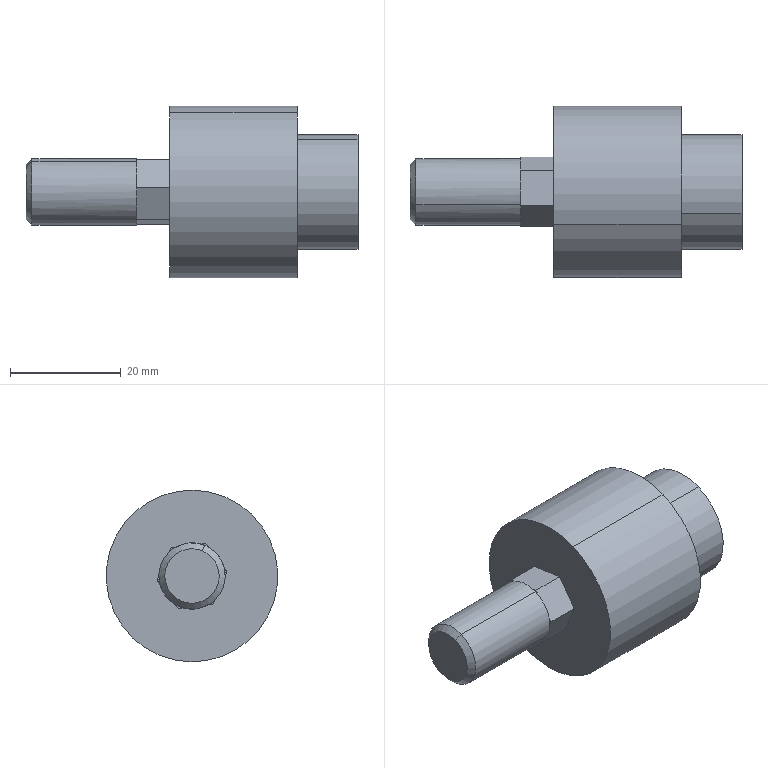Component | SolidWorks | FloatingJointSMCJA40-12-175-1 | 1 solid | 33 faces | box 60 x 31 x 31 mm | volume 22336 mm3 | plane 23 | cylinder 8 | cone 2 | commonest cylinder face diameters 12 x4 31 x2 20.667 x2
STEP:
#1=COLOUR_RGB('',0.7922,0.8196,0.9333);
#2=FILL_AREA_STYLE_COLOUR('',#1);
#3=FILL_AREA_STYLE('',(#2));
#4=SURFACE_STYLE_FILL_AREA(#3);
#5=SURFACE_SIDE_STYLE('',(#4));
#6=SURFACE_STYLE_USAGE(.BOTH.,#5);
#7=PRESENTATION_STYLE_ASSIGNMENT((#6));
#8=CARTESIAN_POINT('',(-1.88,0.09048,-0.2182));
#9=VERTEX_POINT('',#8);
#10=CARTESIAN_POINT('',(-1.88,-0.09048,0.2182));
#11=VERTEX_POINT('',#10);
#12=CARTESIAN_POINT('',(-1.88,-0.,0.));
#13=DIRECTION('',(1.,0.,-0.));
#14=DIRECTION('',(0.,-0.383,0.9237));
#15=AXIS2_PLACEMENT_3D('',#12,#13,#14);
#16=CIRCLE('',#15,0.2362);
#17=EDGE_CURVE('',#9,#11,#16,.T.);
#18=ORIENTED_EDGE('',*,*,#17,.T.);
#19=CARTESIAN_POINT('',(-2.431,-0.09048,0.2182));
#20=VERTEX_POINT('',#19);
#21=CARTESIAN_POINT('',(-1.329,-0.09048,0.2182));
#22=DIRECTION('',(-1.,-0.,0.));
#23=VECTOR('',#22,39.37);
#24=LINE('',#21,#23);
#25=EDGE_CURVE('',#11,#20,#24,.T.);
#26=ORIENTED_EDGE('',*,*,#25,.T.);
#27=CARTESIAN_POINT('',(-2.431,0.09048,-0.2182));
#28=VERTEX_POINT('',#27);
#29=CARTESIAN_POINT('',(-2.431,-0.,0.));
#30=DIRECTION('',(-1.,-0.,0.));
#31=DIRECTION('',(0.,0.383,-0.9237));
#32=AXIS2_PLACEMENT_3D('',#29,#30,#31);
#33=CIRCLE('',#32,0.2362);
#34=EDGE_CURVE('',#20,#28,#33,.T.);
#35=ORIENTED_EDGE('',*,*,#34,.T.);
#36=CARTESIAN_POINT('',(-1.329,0.09048,-0.2182));
#37=DIRECTION('',(-1.,-0.,0.));
#38=VECTOR('',#37,39.37);
#39=LINE('',#36,#38);
#40=EDGE_CURVE('',#9,#28,#39,.T.);
#41=ORIENTED_EDGE('',*,*,#40,.F.);
#42=EDGE_LOOP('',(#18,#26,#35,#41));
#43=FACE_OUTER_BOUND('',#42,.T.);
#44=CARTESIAN_POINT('',(-1.329,0.,-0.));
#45=DIRECTION('',(-1.,-0.,0.));
#46=DIRECTION('',(0.,0.383,-0.9237));
#47=AXIS2_PLACEMENT_3D('',#44,#45,#46);
#48=CYLINDRICAL_SURFACE('',#47,0.2362);
#49=ADVANCED_FACE('',(#43),#48,.F.);
#50=CARTESIAN_POINT('',(-3.219,-0.2338,0.5637));
#51=VERTEX_POINT('',#50);
#52=CARTESIAN_POINT('',(-3.219,0.2338,-0.5637));
#53=VERTEX_POINT('',#52);
#54=CARTESIAN_POINT('',(-3.219,-0.,0.));
#55=DIRECTION('',(1.,0.,-0.));
#56=DIRECTION('',(0.,-0.383,0.9237));
#57=AXIS2_PLACEMENT_3D('',#54,#55,#56);
#58=CIRCLE('',#57,0.6102);
#59=EDGE_CURVE('',#51,#53,#58,.T.);
#60=ORIENTED_EDGE('',*,*,#59,.T.);
#61=CARTESIAN_POINT('',(-2.313,0.2338,-0.5637));
#62=VERTEX_POINT('',#61);
#63=CARTESIAN_POINT('',(-2.766,0.2338,-0.5637));
#64=DIRECTION('',(1.,0.,-0.));
#65=VECTOR('',#64,39.37);
#66=LINE('',#63,#65);
#67=EDGE_CURVE('',#53,#62,#66,.T.);
#68=ORIENTED_EDGE('',*,*,#67,.T.);
#69=CARTESIAN_POINT('',(-2.313,-0.2338,0.5637));
#70=VERTEX_POINT('',#69);
#71=CARTESIAN_POINT('',(-2.313,-0.,0.));
#72=DIRECTION('',(-1.,-0.,0.));
#73=DIRECTION('',(0.,-0.383,0.9237));
#74=AXIS2_PLACEMENT_3D('',#71,#72,#73);
#75=CIRCLE('',#74,0.6102);
#76=EDGE_CURVE('',#62,#70,#75,.T.);
#77=ORIENTED_EDGE('',*,*,#76,.T.);
#78=CARTESIAN_POINT('',(-2.766,-0.2338,0.5637));
#79=DIRECTION('',(1.,0.,-0.));
#80=VECTOR('',#79,39.37);
#81=LINE('',#78,#80);
#82=EDGE_CURVE('',#51,#70,#81,.T.);
#83=ORIENTED_EDGE('',*,*,#82,.F.);
#84=EDGE_LOOP('',(#60,#68,#77,#83));
#85=FACE_OUTER_BOUND('',#84,.T.);
#86=CARTESIAN_POINT('',(-2.766,-0.,0.));
#87=DIRECTION('',(1.,0.,-0.));
#88=DIRECTION('',(0.,-0.383,0.9237));
#89=AXIS2_PLACEMENT_3D('',#86,#87,#88);
#90=CYLINDRICAL_SURFACE('',#89,0.6102);
#91=ADVANCED_FACE('',(#85),#90,.T.);
#92=CARTESIAN_POINT('',(-2.313,0.1558,-0.3758));
#93=VERTEX_POINT('',#92);
#94=CARTESIAN_POINT('',(-2.313,-0.1558,0.3758));
#95=VERTEX_POINT('',#94);
#96=CARTESIAN_POINT('',(-2.313,-0.,0.));
#97=DIRECTION('',(-1.,-0.,0.));
#98=DIRECTION('',(0.,-0.383,0.9237));
#99=AXIS2_PLACEMENT_3D('',#96,#97,#98);
#100=CIRCLE('',#99,0.4068);
#101=EDGE_CURVE('',#93,#95,#100,.T.);
#102=ORIENTED_EDGE('',*,*,#101,.F.);
#103=CARTESIAN_POINT('',(-1.88,0.1558,-0.3758));
#104=VERTEX_POINT('',#103);
#105=CARTESIAN_POINT('',(-2.096,0.1558,-0.3758));
#106=DIRECTION('',(1.,0.,-0.));
#107=VECTOR('',#106,39.37);
#108=LINE('',#105,#107);
#109=EDGE_CURVE('',#93,#104,#108,.T.);
#110=ORIENTED_EDGE('',*,*,#109,.T.);
#111=CARTESIAN_POINT('',(-1.88,-0.1558,0.3758));
#112=VERTEX_POINT('',#111);
#113=CARTESIAN_POINT('',(-1.88,-0.,0.));
#114=DIRECTION('',(-1.,-0.,0.));
#115=DIRECTION('',(0.,-0.383,0.9237));
#116=AXIS2_PLACEMENT_3D('',#113,#114,#115);
#117=CIRCLE('',#116,0.4068);
#118=EDGE_CURVE('',#104,#112,#117,.T.);
#119=ORIENTED_EDGE('',*,*,#118,.T.);
#120=CARTESIAN_POINT('',(-2.096,-0.1558,0.3758));
#121=DIRECTION('',(1.,0.,-0.));
#122=VECTOR('',#121,39.37);
#123=LINE('',#120,#122);
#124=EDGE_CURVE('',#95,#112,#123,.T.);
#125=ORIENTED_EDGE('',*,*,#124,.F.);
#126=EDGE_LOOP('',(#102,#110,#119,#125));
#127=FACE_OUTER_BOUND('',#126,.T.);
#128=CARTESIAN_POINT('',(-2.096,-0.,0.));
#129=DIRECTION('',(1.,0.,-0.));
#130=DIRECTION('',(0.,-0.383,0.9237));
#131=AXIS2_PLACEMENT_3D('',#128,#129,#130);
#132=CYLINDRICAL_SURFACE('',#131,0.4068);
#133=ADVANCED_FACE('',(#127),#132,.T.);
#134=CARTESIAN_POINT('',(-4.2,-0.09048,0.2182));
#135=VERTEX_POINT('',#134);
#136=CARTESIAN_POINT('',(-4.2,0.09048,-0.2182));
#137=VERTEX_POINT('',#136);
#138=CARTESIAN_POINT('',(-4.2,-0.,0.));
#139=DIRECTION('',(1.,0.,-0.));
#140=DIRECTION('',(0.,-0.383,0.9237));
#141=AXIS2_PLACEMENT_3D('',#138,#139,#140);
#142=CIRCLE('',#141,0.2362);
#143=EDGE_CURVE('',#135,#137,#142,.T.);
#144=ORIENTED_EDGE('',*,*,#143,.T.);
#145=CARTESIAN_POINT('',(-3.455,0.09048,-0.2182));
#146=VERTEX_POINT('',#145);
#147=CARTESIAN_POINT('',(-3.827,0.09048,-0.2182));
#148=DIRECTION('',(1.,0.,-0.));
#149=VECTOR('',#148,39.37);
#150=LINE('',#147,#149);
#151=EDGE_CURVE('',#137,#146,#150,.T.);
#152=ORIENTED_EDGE('',*,*,#151,.T.);
#153=CARTESIAN_POINT('',(-3.455,0.06542,-0.227));
#154=VERTEX_POINT('',#153);
#155=CARTESIAN_POINT('',(-3.455,-0.,0.));
#156=DIRECTION('',(1.,0.,-0.));
#157=DIRECTION('',(0.,-0.383,0.9237));
#158=AXIS2_PLACEMENT_3D('',#155,#156,#157);
#159=CIRCLE('',#158,0.2362);
#160=EDGE_CURVE('',#154,#146,#159,.T.);
#161=ORIENTED_EDGE('',*,*,#160,.F.);
#162=CARTESIAN_POINT('',(-3.455,-0.1218,-0.2024));
#163=VERTEX_POINT('',#162);
#164=CARTESIAN_POINT('',(-3.455,-0.,0.));
#165=DIRECTION('',(1.,0.,-0.));
#166=DIRECTION('',(0.,-0.383,0.9237));
#167=AXIS2_PLACEMENT_3D('',#164,#165,#166);
#168=CIRCLE('',#167,0.2362);
#169=EDGE_CURVE('',#163,#154,#168,.T.);
#170=ORIENTED_EDGE('',*,*,#169,.F.);
#171=CARTESIAN_POINT('',(-3.455,-0.1639,-0.1701));
#172=VERTEX_POINT('',#171);
#173=CARTESIAN_POINT('',(-3.455,-0.,0.));
#174=DIRECTION('',(1.,0.,-0.));
#175=DIRECTION('',(0.,-0.383,0.9237));
#176=AXIS2_PLACEMENT_3D('',#173,#174,#175);
#177=CIRCLE('',#176,0.2362);
#178=EDGE_CURVE('',#172,#163,#177,.T.);
#179=ORIENTED_EDGE('',*,*,#178,.F.);
#180=CARTESIAN_POINT('',(-3.455,-0.2362,0.004262));
#181=VERTEX_POINT('',#180);
#182=CARTESIAN_POINT('',(-3.455,-0.,0.));
#183=DIRECTION('',(1.,0.,-0.));
#184=DIRECTION('',(0.,-0.383,0.9237));
#185=AXIS2_PLACEMENT_3D('',#182,#183,#184);
#186=CIRCLE('',#185,0.2362);
#187=EDGE_CURVE('',#181,#172,#186,.T.);
#188=ORIENTED_EDGE('',*,*,#187,.F.);
#189=CARTESIAN_POINT('',(-3.455,-0.2293,0.05683));
#190=VERTEX_POINT('',#189);
#191=CARTESIAN_POINT('',(-3.455,-0.,0.));
#192=DIRECTION('',(1.,0.,-0.));
#193=DIRECTION('',(0.,-0.383,0.9237));
#194=AXIS2_PLACEMENT_3D('',#191,#192,#193);
#195=CIRCLE('',#194,0.2362);
#196=EDGE_CURVE('',#190,#181,#195,.T.);
#197=ORIENTED_EDGE('',*,*,#196,.F.);
#198=CARTESIAN_POINT('',(-3.455,-0.1144,0.2067));
#199=VERTEX_POINT('',#198);
#200=CARTESIAN_POINT('',(-3.455,-0.,0.));
#201=DIRECTION('',(1.,0.,-0.));
#202=DIRECTION('',(0.,-0.383,0.9237));
#203=AXIS2_PLACEMENT_3D('',#200,#201,#202);
#204=CIRCLE('',#203,0.2362);
#205=EDGE_CURVE('',#199,#190,#204,.T.);
#206=ORIENTED_EDGE('',*,*,#205,.F.);
#207=CARTESIAN_POINT('',(-3.455,-0.09048,0.2182));
#208=VERTEX_POINT('',#207);
#209=CARTESIAN_POINT('',(-3.455,-0.,0.));
#210=DIRECTION('',(1.,0.,-0.));
#211=DIRECTION('',(0.,-0.383,0.9237));
#212=AXIS2_PLACEMENT_3D('',#209,#210,#211);
#213=CIRCLE('',#212,0.2362);
#214=EDGE_CURVE('',#208,#199,#213,.T.);
#215=ORIENTED_EDGE('',*,*,#214,.F.);
#216=CARTESIAN_POINT('',(-3.827,-0.09048,0.2182));
#217=DIRECTION('',(1.,0.,-0.));
#218=VECTOR('',#217,39.37);
#219=LINE('',#216,#218);
#220=EDGE_CURVE('',#135,#208,#219,.T.);
#221=ORIENTED_EDGE('',*,*,#220,.F.);
#222=EDGE_LOOP('',(#144,#152,#161,#170,#179,#188,#197,#206,#215,#221));
#223=FACE_OUTER_BOUND('',#222,.T.);
#224=CARTESIAN_POINT('',(-3.827,-0.,0.));
#225=DIRECTION('',(1.,0.,-0.));
#226=DIRECTION('',(0.,-0.383,0.9237));
#227=AXIS2_PLACEMENT_3D('',#224,#225,#226);
#228=CYLINDRICAL_SURFACE('',#227,0.2362);
#229=ADVANCED_FACE('',(#223),#228,.T.);
#230=CARTESIAN_POINT('',(-4.242,-0.07427,0.1791));
#231=VERTEX_POINT('',#230);
#232=CARTESIAN_POINT('',(-4.242,0.07427,-0.1791));
#233=VERTEX_POINT('',#232);
#234=CARTESIAN_POINT('',(-4.242,-0.,0.));
#235=DIRECTION('',(1.,0.,-0.));
#236=DIRECTION('',(0.,-0.383,0.9237));
#237=AXIS2_PLACEMENT_3D('',#234,#235,#236);
#238=CIRCLE('',#237,0.1939);
#239=EDGE_CURVE('',#231,#233,#238,.T.);
#240=ORIENTED_EDGE('',*,*,#239,.T.);
#241=CARTESIAN_POINT('',(-4.2,0.09048,-0.2182));
#242=DIRECTION('',(0.7071,0.2709,-0.6532));
#243=VECTOR('',#242,39.37);
#244=LINE('',#241,#243);
#245=EDGE_CURVE('',#233,#137,#244,.T.);
#246=ORIENTED_EDGE('',*,*,#245,.T.);
#247=ORIENTED_EDGE('',*,*,#143,.F.);
#248=CARTESIAN_POINT('',(-4.2,-0.09048,0.2182));
#249=DIRECTION('',(0.7071,-0.2709,0.6532));
#250=VECTOR('',#249,39.37);
#251=LINE('',#248,#250);
#252=EDGE_CURVE('',#231,#135,#251,.T.);
#253=ORIENTED_EDGE('',*,*,#252,.F.);
#254=EDGE_LOOP('',(#240,#246,#247,#253));
#255=FACE_OUTER_BOUND('',#254,.T.);
#256=CARTESIAN_POINT('',(-4.2,-0.,0.));
#257=DIRECTION('',(1.,0.,-0.));
#258=DIRECTION('',(0.,-0.383,0.9237));
#259=AXIS2_PLACEMENT_3D('',#256,#257,#258);
#260=CONICAL_SURFACE('',#259,0.2362,0.7854);
#261=ADVANCED_FACE('',(#255),#260,.T.);
#262=ORIENTED_EDGE('',*,*,#67,.F.);
#263=CARTESIAN_POINT('',(-3.219,-0.,0.));
#264=DIRECTION('',(1.,0.,-0.));
#265=DIRECTION('',(0.,-0.383,0.9237));
#266=AXIS2_PLACEMENT_3D('',#263,#264,#265);
#267=CIRCLE('',#266,0.6102);
#268=EDGE_CURVE('',#53,#51,#267,.T.);
#269=ORIENTED_EDGE('',*,*,#268,.T.);
#270=ORIENTED_EDGE('',*,*,#82,.T.);
#271=CARTESIAN_POINT('',(-2.313,-0.,0.));
#272=DIRECTION('',(-1.,-0.,0.));
#273=DIRECTION('',(0.,-0.383,0.9237));
#274=AXIS2_PLACEMENT_3D('',#271,#272,#273);
#275=CIRCLE('',#274,0.6102);
#276=EDGE_CURVE('',#70,#62,#275,.T.);
#277=ORIENTED_EDGE('',*,*,#276,.T.);
#278=EDGE_LOOP('',(#262,#269,#270,#277));
#279=FACE_OUTER_BOUND('',#278,.T.);
#280=CARTESIAN_POINT('',(-2.766,-0.,0.));
#281=DIRECTION('',(1.,0.,-0.));
#282=DIRECTION('',(0.,-0.383,0.9237));
#283=AXIS2_PLACEMENT_3D('',#280,#281,#282);
#284=CYLINDRICAL_SURFACE('',#283,0.6102);
#285=ADVANCED_FACE('',(#279),#284,.T.);
#286=ORIENTED_EDGE('',*,*,#59,.F.);
#287=ORIENTED_EDGE('',*,*,#268,.F.);
#288=EDGE_LOOP('',(#286,#287));
#289=FACE_OUTER_BOUND('',#288,.T.);
#290=CARTESIAN_POINT('',(-3.219,0.09578,-0.231));
#291=VERTEX_POINT('',#290);
#292=CARTESIAN_POINT('',(-3.219,0.2479,-0.03254));
#293=VERTEX_POINT('',#292);
#294=CARTESIAN_POINT('',(-3.219,0.09578,-0.231));
#295=DIRECTION('',(0.,0.6084,0.7936));
#296=VECTOR('',#295,39.37);
#297=LINE('',#294,#296);
#298=EDGE_CURVE('',#291,#293,#297,.T.);
#299=ORIENTED_EDGE('',*,*,#298,.T.);
#300=CARTESIAN_POINT('',(-3.219,0.1521,0.1984));
#301=VERTEX_POINT('',#300);
#302=CARTESIAN_POINT('',(-3.219,0.2,0.08294));
#303=DIRECTION('',(0.,-0.383,0.9237));
#304=VECTOR('',#303,39.37);
#305=LINE('',#302,#304);
#306=EDGE_CURVE('',#293,#301,#305,.T.);
#307=ORIENTED_EDGE('',*,*,#306,.T.);
#308=CARTESIAN_POINT('',(-3.219,-0.09578,0.231));
#309=VERTEX_POINT('',#308);
#310=CARTESIAN_POINT('',(-3.219,0.1521,0.1984));
#311=DIRECTION('',(0.,-0.9915,0.1301));
#312=VECTOR('',#311,39.37);
#313=LINE('',#310,#312);
#314=EDGE_CURVE('',#301,#309,#313,.T.);
#315=ORIENTED_EDGE('',*,*,#314,.T.);
#316=CARTESIAN_POINT('',(-3.219,-0.2479,0.03254));
#317=VERTEX_POINT('',#316);
#318=CARTESIAN_POINT('',(-3.219,-0.09578,0.231));
#319=DIRECTION('',(-0.,-0.6084,-0.7936));
#320=VECTOR('',#319,39.37);
#321=LINE('',#318,#320);
#322=EDGE_CURVE('',#309,#317,#321,.T.);
#323=ORIENTED_EDGE('',*,*,#322,.T.);
#324=CARTESIAN_POINT('',(-3.219,-0.1521,-0.1984));
#325=VERTEX_POINT('',#324);
#326=CARTESIAN_POINT('',(-3.219,-0.2,-0.08294));
#327=DIRECTION('',(-0.,0.383,-0.9237));
#328=VECTOR('',#327,39.37);
#329=LINE('',#326,#328);
#330=EDGE_CURVE('',#317,#325,#329,.T.);
#331=ORIENTED_EDGE('',*,*,#330,.T.);
#332=CARTESIAN_POINT('',(-3.219,-0.1521,-0.1984));
#333=DIRECTION('',(-0.,0.9915,-0.1301));
#334=VECTOR('',#333,39.37);
#335=LINE('',#332,#334);
#336=EDGE_CURVE('',#325,#291,#335,.T.);
#337=ORIENTED_EDGE('',*,*,#336,.T.);
#338=EDGE_LOOP('',(#299,#307,#315,#323,#331,#337));
#339=FACE_BOUND('',#338,.T.);
#340=CARTESIAN_POINT('',(-3.219,-0.2818,-0.1169));
#341=DIRECTION('',(-1.,-0.,0.));
#342=DIRECTION('',(-0.,0.383,-0.9237));
#343=AXIS2_PLACEMENT_3D('',#340,#341,#342);
#344=PLANE('',#343);
#345=ADVANCED_FACE('',(#289,#339),#344,.T.);
#346=CARTESIAN_POINT('',(-2.313,-0.,0.));
#347=DIRECTION('',(-1.,-0.,0.));
#348=DIRECTION('',(0.,-0.383,0.9237));
#349=AXIS2_PLACEMENT_3D('',#346,#347,#348);
#350=CIRCLE('',#349,0.4068);
#351=EDGE_CURVE('',#95,#93,#350,.T.);
#352=ORIENTED_EDGE('',*,*,#351,.T.);
#353=ORIENTED_EDGE('',*,*,#101,.T.);
#354=EDGE_LOOP('',(#352,#353));
#355=FACE_BOUND('',#354,.T.);
#356=ORIENTED_EDGE('',*,*,#276,.F.);
#357=ORIENTED_EDGE('',*,*,#76,.F.);
#358=EDGE_LOOP('',(#356,#357));
#359=FACE_OUTER_BOUND('',#358,.T.);
#360=CARTESIAN_POINT('',(-2.313,-0.4697,-0.1948));
#361=DIRECTION('',(1.,0.,-0.));
#362=DIRECTION('',(0.,-0.383,0.9237));
#363=AXIS2_PLACEMENT_3D('',#360,#361,#362);
#364=PLANE('',#363);
#365=ADVANCED_FACE('',(#355,#359),#364,.T.);
#366=ORIENTED_EDGE('',*,*,#306,.F.);
#367=CARTESIAN_POINT('',(-3.455,0.2479,-0.03254));
#368=VERTEX_POINT('',#367);
#369=CARTESIAN_POINT('',(-3.219,0.2479,-0.03254));
#370=DIRECTION('',(-1.,-0.,0.));
#371=VECTOR('',#370,39.37);
#372=LINE('',#369,#371);
#373=EDGE_CURVE('',#293,#368,#372,.T.);
#374=ORIENTED_EDGE('',*,*,#373,.T.);
#375=CARTESIAN_POINT('',(-3.455,0.2362,-0.004262));
#376=VERTEX_POINT('',#375);
#377=CARTESIAN_POINT('',(-3.455,0.2479,-0.03254));
#378=DIRECTION('',(0.,-0.383,0.9237));
#379=VECTOR('',#378,39.37);
#380=LINE('',#377,#379);
#381=EDGE_CURVE('',#368,#376,#380,.T.);
#382=ORIENTED_EDGE('',*,*,#381,.T.);
#383=CARTESIAN_POINT('',(-3.455,0.1639,0.1701));
#384=VERTEX_POINT('',#383);
#385=CARTESIAN_POINT('',(-3.455,0.2479,-0.03254));
#386=DIRECTION('',(0.,-0.383,0.9237));
#387=VECTOR('',#386,39.37);
#388=LINE('',#385,#387);
#389=EDGE_CURVE('',#376,#384,#388,.T.);
#390=ORIENTED_EDGE('',*,*,#389,.T.);
#391=CARTESIAN_POINT('',(-3.455,0.1521,0.1984));
#392=VERTEX_POINT('',#391);
#393=CARTESIAN_POINT('',(-3.455,0.2479,-0.03254));
#394=DIRECTION('',(0.,-0.383,0.9237));
#395=VECTOR('',#394,39.37);
#396=LINE('',#393,#395);
#397=EDGE_CURVE('',#384,#392,#396,.T.);
#398=ORIENTED_EDGE('',*,*,#397,.T.);
#399=CARTESIAN_POINT('',(-3.219,0.1521,0.1984));
#400=DIRECTION('',(1.,0.,-0.));
#401=VECTOR('',#400,39.37);
#402=LINE('',#399,#401);
#403=EDGE_CURVE('',#392,#301,#402,.T.);
#404=ORIENTED_EDGE('',*,*,#403,.T.);
#405=EDGE_LOOP('',(#366,#374,#382,#390,#398,#404));
#406=FACE_OUTER_BOUND('',#405,.T.);
#407=CARTESIAN_POINT('',(-3.219,0.2479,-0.03254));
#408=DIRECTION('',(-0.,0.9237,0.383));
#409=DIRECTION('',(1.,0.,-0.));
#410=AXIS2_PLACEMENT_3D('',#407,#408,#409);
#411=PLANE('',#410);
#412=ADVANCED_FACE('',(#406),#411,.T.);
#413=ORIENTED_EDGE('',*,*,#298,.F.);
#414=CARTESIAN_POINT('',(-3.455,0.09578,-0.231));
#415=VERTEX_POINT('',#414);
#416=CARTESIAN_POINT('',(-3.219,0.09578,-0.231));
#417=DIRECTION('',(-1.,-0.,0.));
#418=VECTOR('',#417,39.37);
#419=LINE('',#416,#418);
#420=EDGE_CURVE('',#291,#415,#419,.T.);
#421=ORIENTED_EDGE('',*,*,#420,.T.);
#422=CARTESIAN_POINT('',(-3.455,0.1144,-0.2067));
#423=VERTEX_POINT('',#422);
#424=CARTESIAN_POINT('',(-3.455,0.09578,-0.231));
#425=DIRECTION('',(0.,0.6084,0.7936));
#426=VECTOR('',#425,39.37);
#427=LINE('',#424,#426);
#428=EDGE_CURVE('',#415,#423,#427,.T.);
#429=ORIENTED_EDGE('',*,*,#428,.T.);
#430=CARTESIAN_POINT('',(-3.455,0.2293,-0.05683));
#431=VERTEX_POINT('',#430);
#432=CARTESIAN_POINT('',(-3.455,0.09578,-0.231));
#433=DIRECTION('',(0.,0.6084,0.7936));
#434=VECTOR('',#433,39.37);
#435=LINE('',#432,#434);
#436=EDGE_CURVE('',#423,#431,#435,.T.);
#437=ORIENTED_EDGE('',*,*,#436,.T.);
#438=CARTESIAN_POINT('',(-3.455,0.09578,-0.231));
#439=DIRECTION('',(0.,0.6084,0.7936));
#440=VECTOR('',#439,39.37);
#441=LINE('',#438,#440);
#442=EDGE_CURVE('',#431,#368,#441,.T.);
#443=ORIENTED_EDGE('',*,*,#442,.T.);
#444=ORIENTED_EDGE('',*,*,#373,.F.);
#445=EDGE_LOOP('',(#413,#421,#429,#437,#443,#444));
#446=FACE_OUTER_BOUND('',#445,.T.);
#447=CARTESIAN_POINT('',(-3.219,0.09578,-0.231));
#448=DIRECTION('',(-0.,0.7936,-0.6084));
#449=DIRECTION('',(-0.,-0.6084,-0.7936));
#450=AXIS2_PLACEMENT_3D('',#447,#448,#449);
#451=PLANE('',#450);
#452=ADVANCED_FACE('',(#446),#451,.T.);
#453=ORIENTED_EDGE('',*,*,#336,.F.);
#454=CARTESIAN_POINT('',(-3.455,-0.1521,-0.1984));
#455=VERTEX_POINT('',#454);
#456=CARTESIAN_POINT('',(-3.219,-0.1521,-0.1984));
#457=DIRECTION('',(-1.,-0.,0.));
#458=VECTOR('',#457,39.37);
#459=LINE('',#456,#458);
#460=EDGE_CURVE('',#325,#455,#459,.T.);
#461=ORIENTED_EDGE('',*,*,#460,.T.);
#462=CARTESIAN_POINT('',(-3.455,-0.1521,-0.1984));
#463=DIRECTION('',(-0.,0.9915,-0.1301));
#464=VECTOR('',#463,39.37);
#465=LINE('',#462,#464);
#466=EDGE_CURVE('',#455,#163,#465,.T.);
#467=ORIENTED_EDGE('',*,*,#466,.T.);
#468=CARTESIAN_POINT('',(-3.455,-0.1521,-0.1984));
#469=DIRECTION('',(-0.,0.9915,-0.1301));
#470=VECTOR('',#469,39.37);
#471=LINE('',#468,#470);
#472=EDGE_CURVE('',#163,#154,#471,.T.);
#473=ORIENTED_EDGE('',*,*,#472,.T.);
#474=CARTESIAN_POINT('',(-3.455,-0.1521,-0.1984));
#475=DIRECTION('',(-0.,0.9915,-0.1301));
#476=VECTOR('',#475,39.37);
#477=LINE('',#474,#476);
#478=EDGE_CURVE('',#154,#415,#477,.T.);
#479=ORIENTED_EDGE('',*,*,#478,.T.);
#480=ORIENTED_EDGE('',*,*,#420,.F.);
#481=EDGE_LOOP('',(#453,#461,#467,#473,#479,#480));
#482=FACE_OUTER_BOUND('',#481,.T.);
#483=CARTESIAN_POINT('',(-3.219,-0.1521,-0.1984));
#484=DIRECTION('',(-0.,-0.1301,-0.9915));
#485=DIRECTION('',(0.,-0.9915,0.1301));
#486=AXIS2_PLACEMENT_3D('',#483,#484,#485);
#487=PLANE('',#486);
#488=ADVANCED_FACE('',(#482),#487,.T.);
#489=ORIENTED_EDGE('',*,*,#330,.F.);
#490=CARTESIAN_POINT('',(-3.455,-0.2479,0.03254));
#491=VERTEX_POINT('',#490);
#492=CARTESIAN_POINT('',(-3.219,-0.2479,0.03254));
#493=DIRECTION('',(-1.,-0.,0.));
#494=VECTOR('',#493,39.37);
#495=LINE('',#492,#494);
#496=EDGE_CURVE('',#317,#491,#495,.T.);
#497=ORIENTED_EDGE('',*,*,#496,.T.);
#498=CARTESIAN_POINT('',(-3.455,-0.2479,0.03254));
#499=DIRECTION('',(-0.,0.383,-0.9237));
#500=VECTOR('',#499,39.37);
#501=LINE('',#498,#500);
#502=EDGE_CURVE('',#491,#181,#501,.T.);
#503=ORIENTED_EDGE('',*,*,#502,.T.);
#504=CARTESIAN_POINT('',(-3.455,-0.2479,0.03254));
#505=DIRECTION('',(-0.,0.383,-0.9237));
#506=VECTOR('',#505,39.37);
#507=LINE('',#504,#506);
#508=EDGE_CURVE('',#181,#172,#507,.T.);
#509=ORIENTED_EDGE('',*,*,#508,.T.);
#510=CARTESIAN_POINT('',(-3.455,-0.2479,0.03254));
#511=DIRECTION('',(-0.,0.383,-0.9237));
#512=VECTOR('',#511,39.37);
#513=LINE('',#510,#512);
#514=EDGE_CURVE('',#172,#455,#513,.T.);
#515=ORIENTED_EDGE('',*,*,#514,.T.);
#516=ORIENTED_EDGE('',*,*,#460,.F.);
#517=EDGE_LOOP('',(#489,#497,#503,#509,#515,#516));
#518=FACE_OUTER_BOUND('',#517,.T.);
#519=CARTESIAN_POINT('',(-3.219,-0.2479,0.03254));
#520=DIRECTION('',(0.,-0.9237,-0.383));
#521=DIRECTION('',(-1.,-0.,0.));
#522=AXIS2_PLACEMENT_3D('',#519,#520,#521);
#523=PLANE('',#522);
#524=ADVANCED_FACE('',(#518),#523,.T.);
#525=ORIENTED_EDGE('',*,*,#322,.F.);
#526=CARTESIAN_POINT('',(-3.455,-0.09578,0.231));
#527=VERTEX_POINT('',#526);
#528=CARTESIAN_POINT('',(-3.219,-0.09578,0.231));
#529=DIRECTION('',(-1.,-0.,0.));
#530=VECTOR('',#529,39.37);
#531=LINE('',#528,#530);
#532=EDGE_CURVE('',#309,#527,#531,.T.);
#533=ORIENTED_EDGE('',*,*,#532,.T.);
#534=CARTESIAN_POINT('',(-3.455,-0.09578,0.231));
#535=DIRECTION('',(-0.,-0.6084,-0.7936));
#536=VECTOR('',#535,39.37);
#537=LINE('',#534,#536);
#538=EDGE_CURVE('',#527,#199,#537,.T.);
#539=ORIENTED_EDGE('',*,*,#538,.T.);
#540=CARTESIAN_POINT('',(-3.455,-0.09578,0.231));
#541=DIRECTION('',(-0.,-0.6084,-0.7936));
#542=VECTOR('',#541,39.37);
#543=LINE('',#540,#542);
#544=EDGE_CURVE('',#199,#190,#543,.T.);
#545=ORIENTED_EDGE('',*,*,#544,.T.);
#546=CARTESIAN_POINT('',(-3.455,-0.09578,0.231));
#547=DIRECTION('',(-0.,-0.6084,-0.7936));
#548=VECTOR('',#547,39.37);
#549=LINE('',#546,#548);
#550=EDGE_CURVE('',#190,#491,#549,.T.);
#551=ORIENTED_EDGE('',*,*,#550,.T.);
#552=ORIENTED_EDGE('',*,*,#496,.F.);
#553=EDGE_LOOP('',(#525,#533,#539,#545,#551,#552));
#554=FACE_OUTER_BOUND('',#553,.T.);
#555=CARTESIAN_POINT('',(-3.219,-0.09578,0.231));
#556=DIRECTION('',(0.,-0.7936,0.6084));
#557=DIRECTION('',(0.,0.6084,0.7936));
#558=AXIS2_PLACEMENT_3D('',#555,#556,#557);
#559=PLANE('',#558);
#560=ADVANCED_FACE('',(#554),#559,.T.);
#561=ORIENTED_EDGE('',*,*,#314,.F.);
#562=ORIENTED_EDGE('',*,*,#403,.F.);
#563=CARTESIAN_POINT('',(-3.455,0.1218,0.2024));
#564=VERTEX_POINT('',#563);
#565=CARTESIAN_POINT('',(-3.455,0.1521,0.1984));
#566=DIRECTION('',(0.,-0.9915,0.1301));
#567=VECTOR('',#566,39.37);
#568=LINE('',#565,#567);
#569=EDGE_CURVE('',#392,#564,#568,.T.);
#570=ORIENTED_EDGE('',*,*,#569,.T.);
#571=CARTESIAN_POINT('',(-3.455,-0.06542,0.227));
#572=VERTEX_POINT('',#571);
#573=CARTESIAN_POINT('',(-3.455,0.1521,0.1984));
#574=DIRECTION('',(0.,-0.9915,0.1301));
#575=VECTOR('',#574,39.37);
#576=LINE('',#573,#575);
#577=EDGE_CURVE('',#564,#572,#576,.T.);
#578=ORIENTED_EDGE('',*,*,#577,.T.);
#579=CARTESIAN_POINT('',(-3.455,0.1521,0.1984));
#580=DIRECTION('',(0.,-0.9915,0.1301));
#581=VECTOR('',#580,39.37);
#582=LINE('',#579,#581);
#583=EDGE_CURVE('',#572,#527,#582,.T.);
#584=ORIENTED_EDGE('',*,*,#583,.T.);
#585=ORIENTED_EDGE('',*,*,#532,.F.);
#586=EDGE_LOOP('',(#561,#562,#570,#578,#584,#585));
#587=FACE_OUTER_BOUND('',#586,.T.);
#588=CARTESIAN_POINT('',(-3.219,0.1521,0.1984));
#589=DIRECTION('',(0.,0.1301,0.9915));
#590=DIRECTION('',(-0.,0.9915,-0.1301));
#591=AXIS2_PLACEMENT_3D('',#588,#589,#590);
#592=PLANE('',#591);
#593=ADVANCED_FACE('',(#587),#592,.T.);
#594=ORIENTED_EDGE('',*,*,#109,.F.);
#595=ORIENTED_EDGE('',*,*,#351,.F.);
#596=ORIENTED_EDGE('',*,*,#124,.T.);
#597=CARTESIAN_POINT('',(-1.88,-0.,0.));
#598=DIRECTION('',(-1.,-0.,0.));
#599=DIRECTION('',(0.,-0.383,0.9237));
#600=AXIS2_PLACEMENT_3D('',#597,#598,#599);
#601=CIRCLE('',#600,0.4068);
#602=EDGE_CURVE('',#112,#104,#601,.T.);
#603=ORIENTED_EDGE('',*,*,#602,.T.);
#604=EDGE_LOOP('',(#594,#595,#596,#603));
#605=FACE_OUTER_BOUND('',#604,.T.);
#606=CARTESIAN_POINT('',(-2.096,-0.,0.));
#607=DIRECTION('',(1.,0.,-0.));
#608=DIRECTION('',(0.,-0.383,0.9237));
#609=AXIS2_PLACEMENT_3D('',#606,#607,#608);
#610=CYLINDRICAL_SURFACE('',#609,0.4068);
#611=ADVANCED_FACE('',(#605),#610,.T.);
#612=ORIENTED_EDGE('',*,*,#569,.F.);
#613=ORIENTED_EDGE('',*,*,#397,.F.);
#614=CARTESIAN_POINT('',(-3.455,-0.,0.));
#615=DIRECTION('',(-1.,-0.,0.));
#616=DIRECTION('',(0.,-0.383,0.9237));
#617=AXIS2_PLACEMENT_3D('',#614,#615,#616);
#618=CIRCLE('',#617,0.2362);
#619=EDGE_CURVE('',#564,#384,#618,.T.);
#620=ORIENTED_EDGE('',*,*,#619,.F.);
#621=EDGE_LOOP('',(#612,#613,#620));
#622=FACE_OUTER_BOUND('',#621,.T.);
#623=CARTESIAN_POINT('',(-3.455,-0.,0.));
#624=DIRECTION('',(-1.,-0.,0.));
#625=DIRECTION('',(-0.,0.383,-0.9237));
#626=AXIS2_PLACEMENT_3D('',#623,#624,#625);
#627=PLANE('',#626);
#628=ADVANCED_FACE('',(#622),#627,.T.);
#629=ORIENTED_EDGE('',*,*,#389,.F.);
#630=CARTESIAN_POINT('',(-3.455,-0.,0.));
#631=DIRECTION('',(1.,0.,-0.));
#632=DIRECTION('',(0.,-0.383,0.9237));
#633=AXIS2_PLACEMENT_3D('',#630,#631,#632);
#634=CIRCLE('',#633,0.2362);
#635=EDGE_CURVE('',#376,#384,#634,.T.);
#636=ORIENTED_EDGE('',*,*,#635,.T.);
#637=EDGE_LOOP('',(#629,#636));
#638=FACE_OUTER_BOUND('',#637,.T.);
#639=CARTESIAN_POINT('',(-3.455,-0.1091,-0.04524));
#640=DIRECTION('',(1.,0.,-0.));
#641=DIRECTION('',(0.,-0.383,0.9237));
#642=AXIS2_PLACEMENT_3D('',#639,#640,#641);
#643=PLANE('',#642);
#644=ADVANCED_FACE('',(#638),#643,.T.);
#645=ORIENTED_EDGE('',*,*,#381,.F.);
#646=ORIENTED_EDGE('',*,*,#442,.F.);
#647=CARTESIAN_POINT('',(-3.455,-0.,0.));
#648=DIRECTION('',(1.,0.,-0.));
#649=DIRECTION('',(0.,-0.383,0.9237));
#650=AXIS2_PLACEMENT_3D('',#647,#648,#649);
#651=CIRCLE('',#650,0.2362);
#652=EDGE_CURVE('',#431,#376,#651,.T.);
#653=ORIENTED_EDGE('',*,*,#652,.T.);
#654=EDGE_LOOP('',(#645,#646,#653));
#655=FACE_OUTER_BOUND('',#654,.T.);
#656=CARTESIAN_POINT('',(-3.455,-0.,0.));
#657=DIRECTION('',(-1.,-0.,0.));
#658=DIRECTION('',(-0.,0.383,-0.9237));
#659=AXIS2_PLACEMENT_3D('',#656,#657,#658);
#660=PLANE('',#659);
#661=ADVANCED_FACE('',(#655),#660,.T.);
#662=ORIENTED_EDGE('',*,*,#436,.F.);
#663=CARTESIAN_POINT('',(-3.455,-0.,0.));
#664=DIRECTION('',(1.,0.,-0.));
#665=DIRECTION('',(0.,-0.383,0.9237));
#666=AXIS2_PLACEMENT_3D('',#663,#664,#665);
#667=CIRCLE('',#666,0.2362);
#668=EDGE_CURVE('',#423,#431,#667,.T.);
#669=ORIENTED_EDGE('',*,*,#668,.T.);
#670=EDGE_LOOP('',(#662,#669));
#671=FACE_OUTER_BOUND('',#670,.T.);
#672=CARTESIAN_POINT('',(-3.455,-0.1091,-0.04524));
#673=DIRECTION('',(1.,0.,-0.));
#674=DIRECTION('',(0.,-0.383,0.9237));
#675=AXIS2_PLACEMENT_3D('',#672,#673,#674);
#676=PLANE('',#675);
#677=ADVANCED_FACE('',(#671),#676,.T.);
#678=ORIENTED_EDGE('',*,*,#428,.F.);
#679=ORIENTED_EDGE('',*,*,#478,.F.);
#680=ORIENTED_EDGE('',*,*,#160,.T.);
#681=CARTESIAN_POINT('',(-3.455,-0.,0.));
#682=DIRECTION('',(1.,0.,-0.));
#683=DIRECTION('',(0.,-0.383,0.9237));
#684=AXIS2_PLACEMENT_3D('',#681,#682,#683);
#685=CIRCLE('',#684,0.2362);
#686=EDGE_CURVE('',#146,#423,#685,.T.);
#687=ORIENTED_EDGE('',*,*,#686,.T.);
#688=EDGE_LOOP('',(#678,#679,#680,#687));
#689=FACE_OUTER_BOUND('',#688,.T.);
#690=CARTESIAN_POINT('',(-3.455,-0.,0.));
#691=DIRECTION('',(-1.,-0.,0.));
#692=DIRECTION('',(-0.,0.383,-0.9237));
#693=AXIS2_PLACEMENT_3D('',#690,#691,#692);
#694=PLANE('',#693);
#695=ADVANCED_FACE('',(#689),#694,.T.);
#696=ORIENTED_EDGE('',*,*,#472,.F.);
#697=ORIENTED_EDGE('',*,*,#169,.T.);
#698=EDGE_LOOP('',(#696,#697));
#699=FACE_OUTER_BOUND('',#698,.T.);
#700=CARTESIAN_POINT('',(-3.455,-0.1091,-0.04524));
#701=DIRECTION('',(1.,0.,-0.));
#702=DIRECTION('',(0.,-0.383,0.9237));
#703=AXIS2_PLACEMENT_3D('',#700,#701,#702);
#704=PLANE('',#703);
#705=ADVANCED_FACE('',(#699),#704,.T.);
#706=ORIENTED_EDGE('',*,*,#466,.F.);
#707=ORIENTED_EDGE('',*,*,#514,.F.);
#708=ORIENTED_EDGE('',*,*,#178,.T.);
#709=EDGE_LOOP('',(#706,#707,#708));
#710=FACE_OUTER_BOUND('',#709,.T.);
#711=CARTESIAN_POINT('',(-3.455,-0.,0.));
#712=DIRECTION('',(-1.,-0.,0.));
#713=DIRECTION('',(-0.,0.383,-0.9237));
#714=AXIS2_PLACEMENT_3D('',#711,#712,#713);
#715=PLANE('',#714);
#716=ADVANCED_FACE('',(#710),#715,.T.);
#717=ORIENTED_EDGE('',*,*,#508,.F.);
#718=ORIENTED_EDGE('',*,*,#187,.T.);
#719=EDGE_LOOP('',(#717,#718));
#720=FACE_OUTER_BOUND('',#719,.T.);
#721=CARTESIAN_POINT('',(-3.455,-0.1091,-0.04524));
#722=DIRECTION('',(1.,0.,-0.));
#723=DIRECTION('',(0.,-0.383,0.9237));
#724=AXIS2_PLACEMENT_3D('',#721,#722,#723);
#725=PLANE('',#724);
#726=ADVANCED_FACE('',(#720),#725,.T.);
#727=ORIENTED_EDGE('',*,*,#502,.F.);
#728=ORIENTED_EDGE('',*,*,#550,.F.);
#729=ORIENTED_EDGE('',*,*,#196,.T.);
#730=EDGE_LOOP('',(#727,#728,#729));
#731=FACE_OUTER_BOUND('',#730,.T.);
#732=CARTESIAN_POINT('',(-3.455,-0.,0.));
#733=DIRECTION('',(-1.,-0.,0.));
#734=DIRECTION('',(-0.,0.383,-0.9237));
#735=AXIS2_PLACEMENT_3D('',#732,#733,#734);
#736=PLANE('',#735);
#737=ADVANCED_FACE('',(#731),#736,.T.);
#738=ORIENTED_EDGE('',*,*,#544,.F.);
#739=ORIENTED_EDGE('',*,*,#205,.T.);
#740=EDGE_LOOP('',(#738,#739));
#741=FACE_OUTER_BOUND('',#740,.T.);
#742=CARTESIAN_POINT('',(-3.455,-0.1091,-0.04524));
#743=DIRECTION('',(1.,0.,-0.));
#744=DIRECTION('',(0.,-0.383,0.9237));
#745=AXIS2_PLACEMENT_3D('',#742,#743,#744);
#746=PLANE('',#745);
#747=ADVANCED_FACE('',(#741),#746,.T.);
#748=ORIENTED_EDGE('',*,*,#538,.F.);
#749=ORIENTED_EDGE('',*,*,#583,.F.);
#750=CARTESIAN_POINT('',(-3.455,-0.,0.));
#751=DIRECTION('',(1.,0.,-0.));
#752=DIRECTION('',(0.,-0.383,0.9237));
#753=AXIS2_PLACEMENT_3D('',#750,#751,#752);
#754=CIRCLE('',#753,0.2362);
#755=EDGE_CURVE('',#572,#208,#754,.T.);
#756=ORIENTED_EDGE('',*,*,#755,.T.);
#757=ORIENTED_EDGE('',*,*,#214,.T.);
#758=EDGE_LOOP('',(#748,#749,#756,#757));
#759=FACE_OUTER_BOUND('',#758,.T.);
#760=CARTESIAN_POINT('',(-3.455,-0.,0.));
#761=DIRECTION('',(-1.,-0.,0.));
#762=DIRECTION('',(-0.,0.383,-0.9237));
#763=AXIS2_PLACEMENT_3D('',#760,#761,#762);
#764=PLANE('',#763);
#765=ADVANCED_FACE('',(#759),#764,.T.);
#766=ORIENTED_EDGE('',*,*,#577,.F.);
#767=CARTESIAN_POINT('',(-3.455,-0.,0.));
#768=DIRECTION('',(1.,0.,-0.));
#769=DIRECTION('',(0.,-0.383,0.9237));
#770=AXIS2_PLACEMENT_3D('',#767,#768,#769);
#771=CIRCLE('',#770,0.2362);
#772=EDGE_CURVE('',#564,#572,#771,.T.);
#773=ORIENTED_EDGE('',*,*,#772,.T.);
#774=EDGE_LOOP('',(#766,#773));
#775=FACE_OUTER_BOUND('',#774,.T.);
#776=CARTESIAN_POINT('',(-3.455,-0.1091,-0.04524));
#777=DIRECTION('',(1.,0.,-0.));
#778=DIRECTION('',(0.,-0.383,0.9237));
#779=AXIS2_PLACEMENT_3D('',#776,#777,#778);
#780=PLANE('',#779);
#781=ADVANCED_FACE('',(#775),#780,.T.);
#782=ORIENTED_EDGE('',*,*,#17,.F.);
#783=CARTESIAN_POINT('',(-1.88,-0.,0.));
#784=DIRECTION('',(1.,0.,-0.));
#785=DIRECTION('',(0.,-0.383,0.9237));
#786=AXIS2_PLACEMENT_3D('',#783,#784,#785);
#787=CIRCLE('',#786,0.2362);
#788=EDGE_CURVE('',#11,#9,#787,.T.);
#789=ORIENTED_EDGE('',*,*,#788,.F.);
#790=EDGE_LOOP('',(#782,#789));
#791=FACE_BOUND('',#790,.T.);
#792=ORIENTED_EDGE('',*,*,#602,.F.);
#793=ORIENTED_EDGE('',*,*,#118,.F.);
#794=EDGE_LOOP('',(#792,#793));
#795=FACE_OUTER_BOUND('',#794,.T.);
#796=CARTESIAN_POINT('',(-1.88,-0.297,-0.1232));
#797=DIRECTION('',(1.,0.,-0.));
#798=DIRECTION('',(0.,-0.383,0.9237));
#799=AXIS2_PLACEMENT_3D('',#796,#797,#798);
#800=PLANE('',#799);
#801=ADVANCED_FACE('',(#791,#795),#800,.T.);
#802=ORIENTED_EDGE('',*,*,#151,.F.);
#803=CARTESIAN_POINT('',(-4.2,-0.,0.));
#804=DIRECTION('',(1.,0.,-0.));
#805=DIRECTION('',(0.,-0.383,0.9237));
#806=AXIS2_PLACEMENT_3D('',#803,#804,#805);
#807=CIRCLE('',#806,0.2362);
#808=EDGE_CURVE('',#137,#135,#807,.T.);
#809=ORIENTED_EDGE('',*,*,#808,.T.);
#810=ORIENTED_EDGE('',*,*,#220,.T.);
#811=ORIENTED_EDGE('',*,*,#755,.F.);
#812=ORIENTED_EDGE('',*,*,#772,.F.);
#813=ORIENTED_EDGE('',*,*,#619,.T.);
#814=ORIENTED_EDGE('',*,*,#635,.F.);
#815=ORIENTED_EDGE('',*,*,#652,.F.);
#816=ORIENTED_EDGE('',*,*,#668,.F.);
#817=ORIENTED_EDGE('',*,*,#686,.F.);
#818=EDGE_LOOP('',(#802,#809,#810,#811,#812,#813,#814,#815,#816,#817));
#819=FACE_OUTER_BOUND('',#818,.T.);
#820=CARTESIAN_POINT('',(-3.827,-0.,0.));
#821=DIRECTION('',(1.,0.,-0.));
#822=DIRECTION('',(0.,-0.383,0.9237));
#823=AXIS2_PLACEMENT_3D('',#820,#821,#822);
#824=CYLINDRICAL_SURFACE('',#823,0.2362);
#825=ADVANCED_FACE('',(#819),#824,.T.);
#826=ORIENTED_EDGE('',*,*,#245,.F.);
#827=CARTESIAN_POINT('',(-4.242,-0.,0.));
#828=DIRECTION('',(1.,0.,-0.));
#829=DIRECTION('',(0.,-0.383,0.9237));
#830=AXIS2_PLACEMENT_3D('',#827,#828,#829);
#831=CIRCLE('',#830,0.1939);
#832=EDGE_CURVE('',#233,#231,#831,.T.);
#833=ORIENTED_EDGE('',*,*,#832,.T.);
#834=ORIENTED_EDGE('',*,*,#252,.T.);
#835=ORIENTED_EDGE('',*,*,#808,.F.);
#836=EDGE_LOOP('',(#826,#833,#834,#835));
#837=FACE_OUTER_BOUND('',#836,.T.);
#838=CARTESIAN_POINT('',(-4.2,-0.,0.));
#839=DIRECTION('',(1.,0.,-0.));
#840=DIRECTION('',(0.,-0.383,0.9237));
#841=AXIS2_PLACEMENT_3D('',#838,#839,#840);
#842=CONICAL_SURFACE('',#841,0.2362,0.7854);
#843=ADVANCED_FACE('',(#837),#842,.T.);
#844=ORIENTED_EDGE('',*,*,#239,.F.);
#845=ORIENTED_EDGE('',*,*,#832,.F.);
#846=EDGE_LOOP('',(#844,#845));
#847=FACE_OUTER_BOUND('',#846,.T.);
#848=CARTESIAN_POINT('',(-4.242,-0.08955,-0.03714));
#849=DIRECTION('',(-1.,-0.,0.));
#850=DIRECTION('',(-0.,0.383,-0.9237));
#851=AXIS2_PLACEMENT_3D('',#848,#849,#850);
#852=PLANE('',#851);
#853=ADVANCED_FACE('',(#847),#852,.T.);
#854=ORIENTED_EDGE('',*,*,#25,.F.);
#855=ORIENTED_EDGE('',*,*,#788,.T.);
#856=ORIENTED_EDGE('',*,*,#40,.T.);
#857=CARTESIAN_POINT('',(-2.431,-0.,0.));
#858=DIRECTION('',(-1.,-0.,0.));
#859=DIRECTION('',(0.,0.383,-0.9237));
#860=AXIS2_PLACEMENT_3D('',#857,#858,#859);
#861=CIRCLE('',#860,0.2362);
#862=EDGE_CURVE('',#28,#20,#861,.T.);
#863=ORIENTED_EDGE('',*,*,#862,.T.);
#864=EDGE_LOOP('',(#854,#855,#856,#863));
#865=FACE_OUTER_BOUND('',#864,.T.);
#866=CARTESIAN_POINT('',(-1.329,0.,-0.));
#867=DIRECTION('',(-1.,-0.,0.));
#868=DIRECTION('',(0.,0.383,-0.9237));
#869=AXIS2_PLACEMENT_3D('',#866,#867,#868);
#870=CYLINDRICAL_SURFACE('',#869,0.2362);
#871=ADVANCED_FACE('',(#865),#870,.F.);
#872=ORIENTED_EDGE('',*,*,#862,.F.);
#873=ORIENTED_EDGE('',*,*,#34,.F.);
#874=EDGE_LOOP('',(#872,#873));
#875=FACE_OUTER_BOUND('',#874,.T.);
#876=CARTESIAN_POINT('',(-2.431,-0.,0.));
#877=DIRECTION('',(-1.,-0.,0.));
#878=DIRECTION('',(-0.,0.383,-0.9237));
#879=AXIS2_PLACEMENT_3D('',#876,#877,#878);
#880=PLANE('',#879);
#881=ADVANCED_FACE('',(#875),#880,.F.);
#882=CLOSED_SHELL('',(#49,#91,#133,#229,#261,#285,#345,#365,#412,#452,#488,#524,#560,#593,#611,#628,#644,#661,#677,#695,#705,#716,#726,#737,#747,#765,#781,#801,#825,#843,#853,#871,#881));
#883=MANIFOLD_SOLID_BREP('',#882);
#884=STYLED_ITEM('',(#7),#883);
#885=(LENGTH_UNIT()NAMED_UNIT(*)SI_UNIT($,.METRE.));
#886=LENGTH_MEASURE_WITH_UNIT(LENGTH_MEASURE(0.0254),#885);
#887=DIMENSIONAL_EXPONENTS(1.,0.,0.,0.,0.,0.,0.);
#888=(CONVERSION_BASED_UNIT('',#886)LENGTH_UNIT()NAMED_UNIT(#887));
#889=UNCERTAINTY_MEASURE_WITH_UNIT(LENGTH_MEASURE(0.00001),#888,'','');
#890=(NAMED_UNIT(*)PLANE_ANGLE_UNIT()SI_UNIT($,.RADIAN.));
#891=(NAMED_UNIT(*)SI_UNIT($,.STERADIAN.)SOLID_ANGLE_UNIT());
#892=(GEOMETRIC_REPRESENTATION_CONTEXT(3)GLOBAL_UNCERTAINTY_ASSIGNED_CONTEXT((#889))GLOBAL_UNIT_ASSIGNED_CONTEXT((#888,#890,#891))REPRESENTATION_CONTEXT('',''));
#893=MECHANICAL_DESIGN_GEOMETRIC_PRESENTATION_REPRESENTATION('',(#884),#892);
#894=PRESENTATION_LAYER_ASSIGNMENT('','',(#884));
#895=CARTESIAN_POINT('',(0.,0.,0.));
#896=DIRECTION('',(0.,0.,1.));
#897=DIRECTION('',(1.,0.,0.));
#898=AXIS2_PLACEMENT_3D('',#895,#896,#897);
#899=(LENGTH_UNIT()NAMED_UNIT(*)SI_UNIT($,.METRE.));
#900=LENGTH_MEASURE_WITH_UNIT(LENGTH_MEASURE(0.0254),#899);
#901=DIMENSIONAL_EXPONENTS(1.,0.,0.,0.,0.,0.,0.);
#902=(CONVERSION_BASED_UNIT('',#900)LENGTH_UNIT()NAMED_UNIT(#901));
#903=UNCERTAINTY_MEASURE_WITH_UNIT(LENGTH_MEASURE(0.00001),#902,'','');
#904=(NAMED_UNIT(*)PLANE_ANGLE_UNIT()SI_UNIT($,.RADIAN.));
#905=(NAMED_UNIT(*)SI_UNIT($,.STERADIAN.)SOLID_ANGLE_UNIT());
#906=(GEOMETRIC_REPRESENTATION_CONTEXT(3)GLOBAL_UNCERTAINTY_ASSIGNED_CONTEXT((#903))GLOBAL_UNIT_ASSIGNED_CONTEXT((#902,#904,#905))REPRESENTATION_CONTEXT('',''));
#907=ADVANCED_BREP_SHAPE_REPRESENTATION('',(#883,#898),#906);